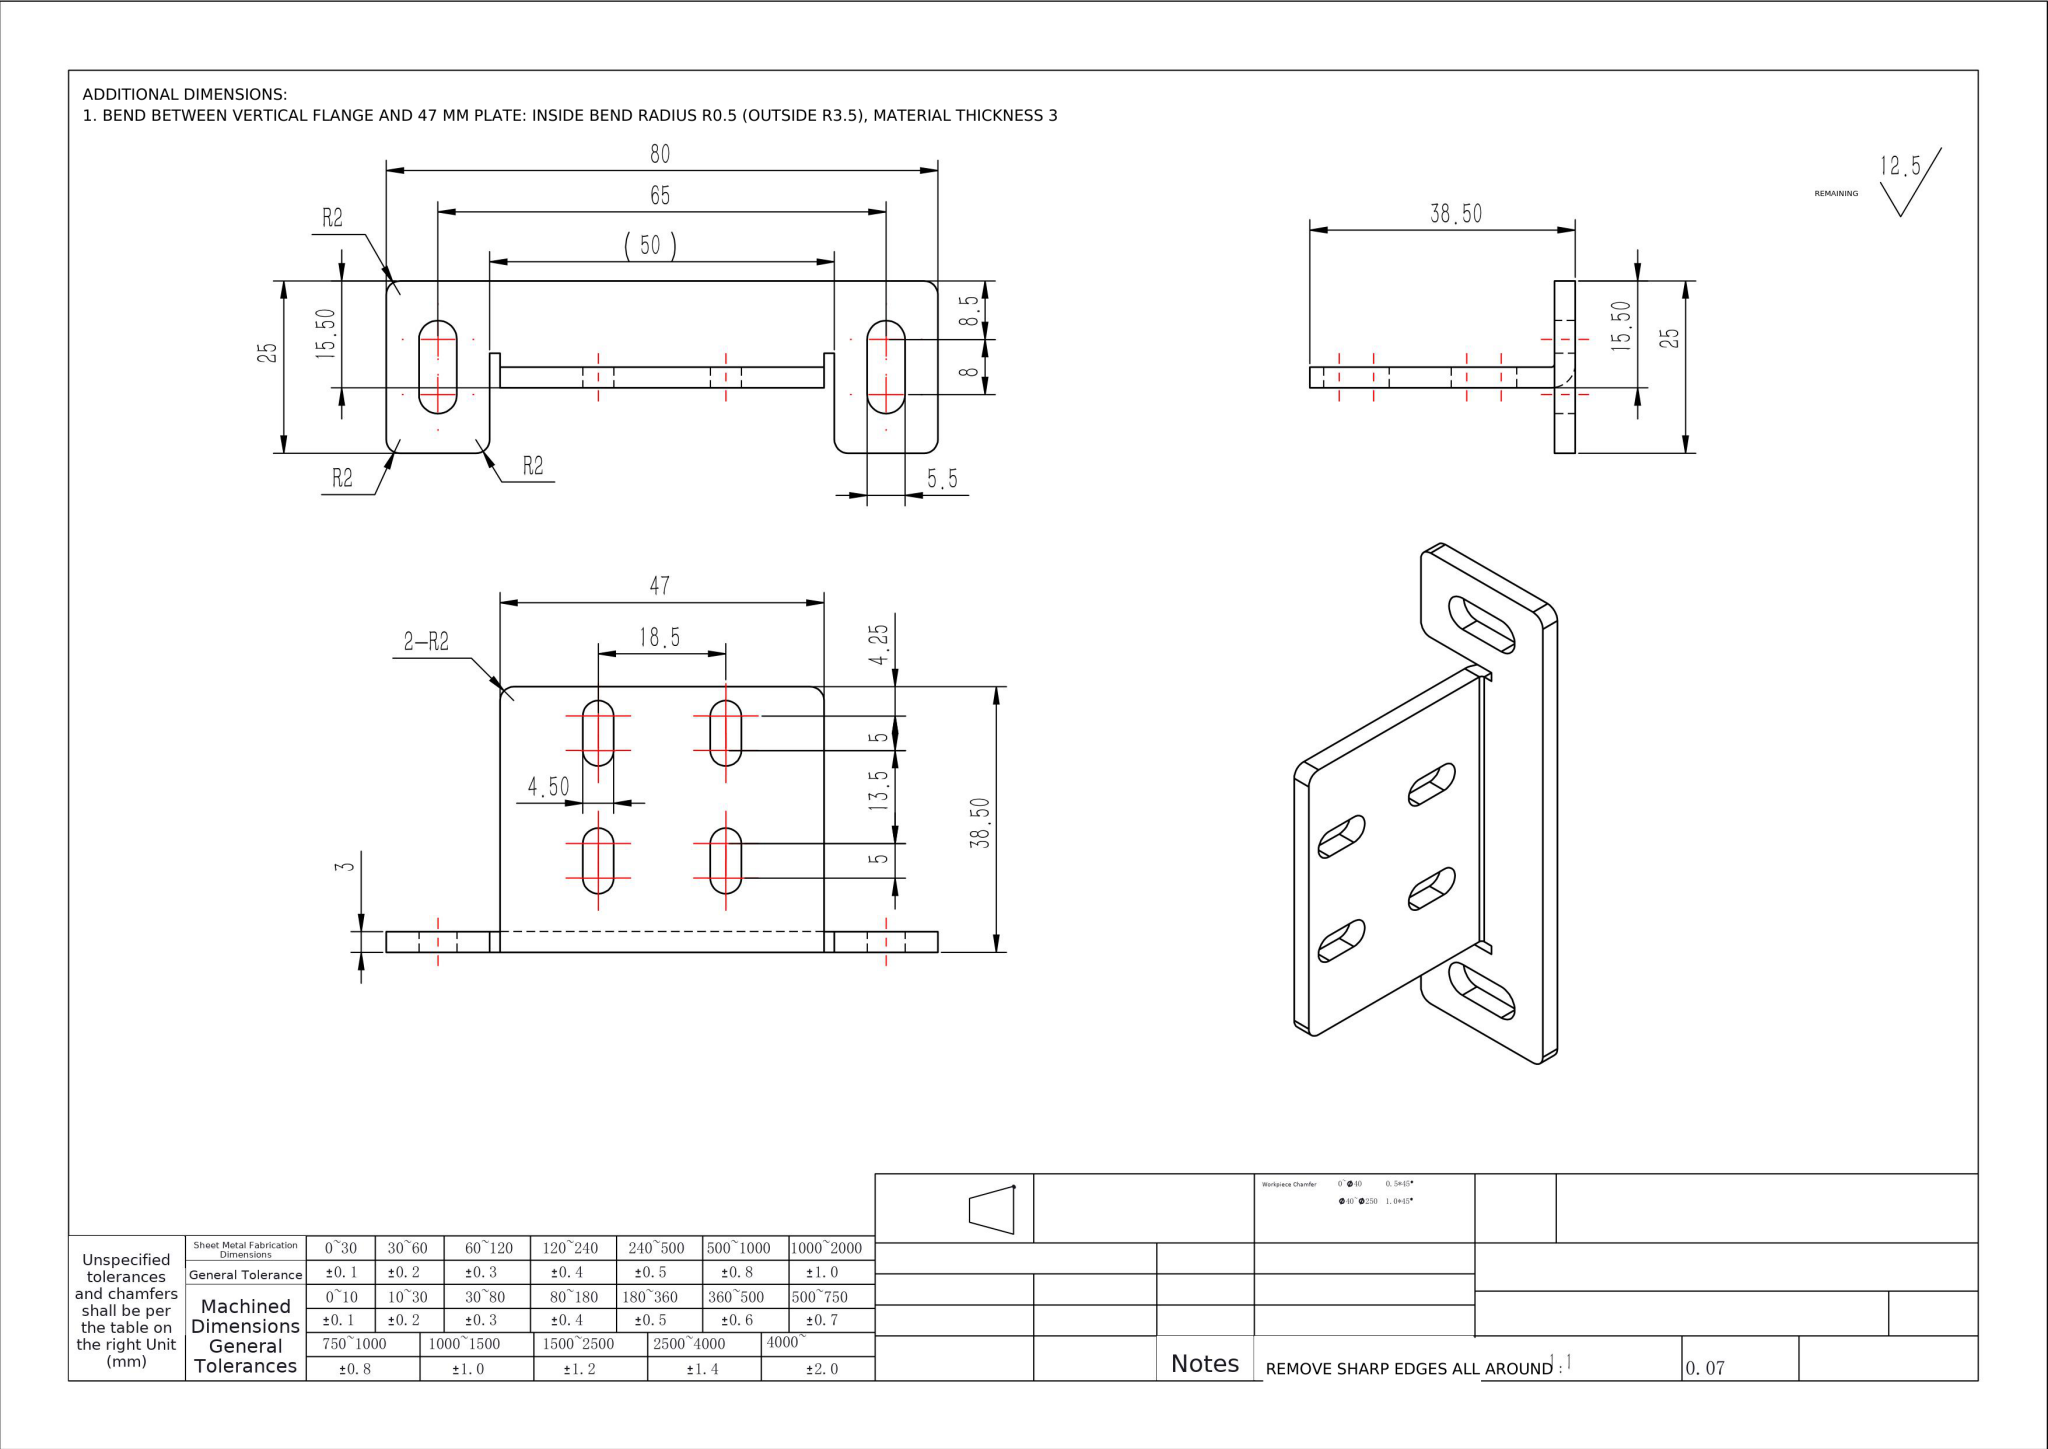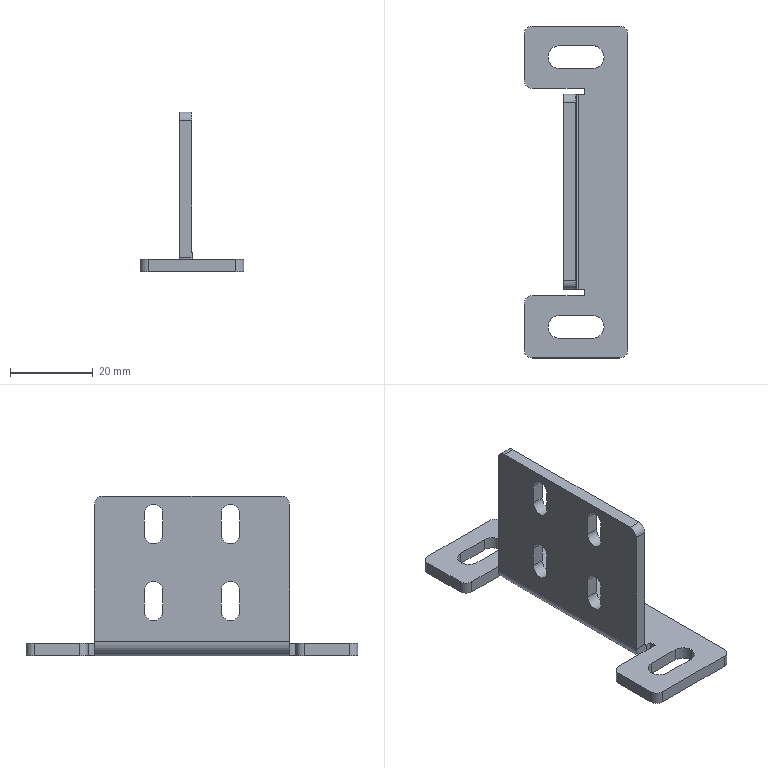Part | NX | mm | 1 solid | 60 faces | box 25 x 80 x 38.5 mm | volume 8526 mm3 | plane 32 | cylinder 28 | commonest cylinder face diameters 4.5 x12 4 x8 5.5 x6 7 x1 1 x1